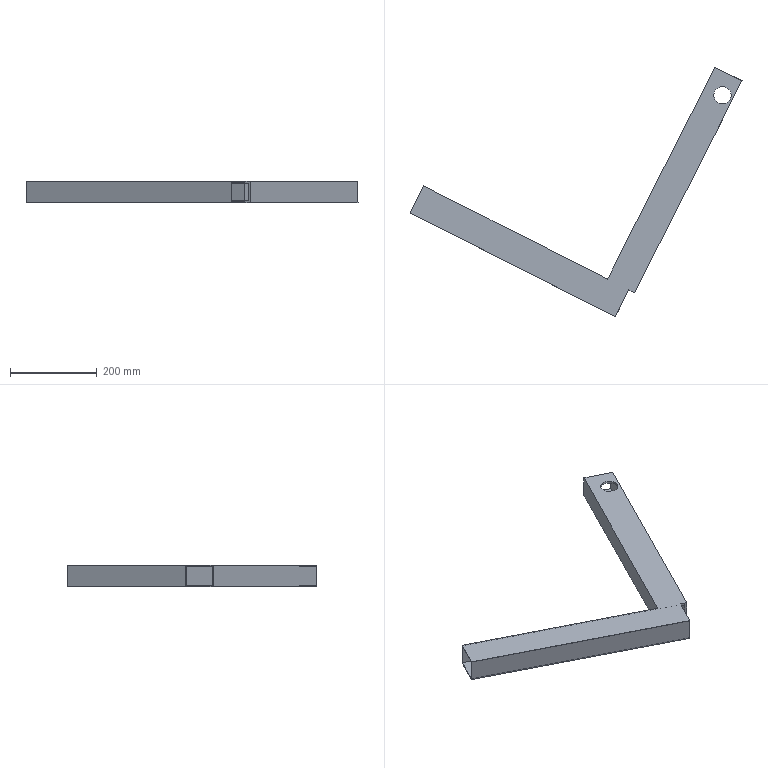Component | SolidWorks | FrameAssemblyDrawing11111-1_Part6-1 | 1 solid | 23 faces | box 765.52 x 576.1 x 50 mm | volume 836154 mm3 | plane 19 | cylinder 4 | commonest cylinder face diameters 40 x4
build123d program:
from build123d import *

# Parameters (mm, degrees)
SKETCH1_W           = 530
SKETCH1_H           = 70
BOSS_EXTRUDE1_DEPTH = 50
SHELL1_T            = -2
SKETCH2_W           = 50
SKETCH2_H           = 70
SKETCH2_W_2         = 40
SKETCH2_H_2         = 60
BOSS_EXTRUDE2_DEPTH = 548
SKETCH3_R           = 20
CUT_EXTRUDE1_DEPTH  = 779.905


with BuildPart() as part:
    # Sketch1 → Boss-Extrude1 (new body)
    with BuildSketch(Plane(origin=(0, 0, 0), x_dir=(0, 0, -1), z_dir=(1, 0, 0))):
        with Locations((198.067, 29.899)):
            Rectangle(SKETCH1_W, SKETCH1_H)
    extrude(amount=BOSS_EXTRUDE1_DEPTH)

    # Shell1
    shell1_openings = [part.faces().sort_by_distance(p)[0] for p in [
        (25, 29.899, -463.067),
        (25, 29.899, 66.933),
    ]]
    offset(amount=SHELL1_T, openings=shell1_openings, kind=Kind.INTERSECTION)

    # Sketch2 → Boss-Extrude2 (add)
    with BuildSketch(Plane(origin=(0, 64.899, 0), x_dir=(1, 0, 0), z_dir=(0, 1, 0))):
        with Locations((25, 443.067)):
            Rectangle(SKETCH2_W, SKETCH2_H)
        with Locations((25, 443.067)):
            Rectangle(SKETCH2_W_2, SKETCH2_H_2, mode=Mode.SUBTRACT)
    extrude(amount=BOSS_EXTRUDE2_DEPTH)

    # Sketch3 → Cut-Extrude1 (cut, through all)
    with BuildSketch(Plane(origin=(50, 0, 0), x_dir=(0, 0, -1), z_dir=(1, 0, 0))):
        with Locations((453.067, 562.899)):
            Circle(SKETCH3_R)
    extrude(amount=-CUT_EXTRUDE1_DEPTH, mode=Mode.SUBTRACT)


solid = part.part

# Placed as in the assembly
solid = solid.moved(Location((-784.566, -450.583, 1035.971), (-90, -63.121, -90)))
STEP:
#1=COLOUR_RGB('',0.7922,0.8196,0.9333);
#2=FILL_AREA_STYLE_COLOUR('',#1);
#3=FILL_AREA_STYLE('',(#2));
#4=SURFACE_STYLE_FILL_AREA(#3);
#5=SURFACE_SIDE_STYLE('',(#4));
#6=SURFACE_STYLE_USAGE(.BOTH.,#5);
#7=PRESENTATION_STYLE_ASSIGNMENT((#6));
#8=CARTESIAN_POINT('',(-5.661,-5.681,40.786));
#9=VERTEX_POINT('',#8);
#10=CARTESIAN_POINT('',(-4.257,-6.392,40.786));
#11=VERTEX_POINT('',#10);
#12=CARTESIAN_POINT('',(-4.959,-6.036,40.786));
#13=DIRECTION('',(-0.,-0.,1.));
#14=DIRECTION('',(0.892,-0.4521,-0.));
#15=AXIS2_PLACEMENT_3D('',#12,#13,#14);
#16=CIRCLE('',#15,0.7874);
#17=EDGE_CURVE('',#9,#11,#16,.T.);
#18=ORIENTED_EDGE('',*,*,#17,.F.);
#19=CARTESIAN_POINT('',(-5.661,-5.681,40.983));
#20=VERTEX_POINT('',#19);
#21=CARTESIAN_POINT('',(-5.661,-5.681,40.786));
#22=DIRECTION('',(-0.,-0.,1.));
#23=VECTOR('',#22,39.37);
#24=LINE('',#21,#23);
#25=EDGE_CURVE('',#9,#20,#24,.T.);
#26=ORIENTED_EDGE('',*,*,#25,.T.);
#27=CARTESIAN_POINT('',(-4.257,-6.392,40.983));
#28=VERTEX_POINT('',#27);
#29=CARTESIAN_POINT('',(-4.959,-6.036,40.983));
#30=DIRECTION('',(-0.,-0.,1.));
#31=DIRECTION('',(0.892,-0.4521,-0.));
#32=AXIS2_PLACEMENT_3D('',#29,#30,#31);
#33=CIRCLE('',#32,0.7874);
#34=EDGE_CURVE('',#20,#28,#33,.T.);
#35=ORIENTED_EDGE('',*,*,#34,.T.);
#36=CARTESIAN_POINT('',(-4.257,-6.392,40.786));
#37=DIRECTION('',(-0.,-0.,1.));
#38=VECTOR('',#37,39.37);
#39=LINE('',#36,#38);
#40=EDGE_CURVE('',#11,#28,#39,.T.);
#41=ORIENTED_EDGE('',*,*,#40,.F.);
#42=EDGE_LOOP('',(#18,#26,#35,#41));
#43=FACE_OUTER_BOUND('',#42,.T.);
#44=CARTESIAN_POINT('',(-4.959,-6.036,40.786));
#45=DIRECTION('',(-0.,-0.,1.));
#46=DIRECTION('',(0.892,-0.4521,-0.));
#47=AXIS2_PLACEMENT_3D('',#44,#45,#46);
#48=CYLINDRICAL_SURFACE('',#47,0.7874);
#49=ADVANCED_FACE('',(#43),#48,.F.);
#50=CARTESIAN_POINT('',(-4.257,-6.392,42.558));
#51=VERTEX_POINT('',#50);
#52=CARTESIAN_POINT('',(-5.661,-5.681,42.558));
#53=VERTEX_POINT('',#52);
#54=CARTESIAN_POINT('',(-4.959,-6.036,42.558));
#55=DIRECTION('',(0.,0.,-1.));
#56=DIRECTION('',(-0.892,0.4521,0.));
#57=AXIS2_PLACEMENT_3D('',#54,#55,#56);
#58=CIRCLE('',#57,0.7874);
#59=EDGE_CURVE('',#51,#53,#58,.T.);
#60=ORIENTED_EDGE('',*,*,#59,.T.);
#61=CARTESIAN_POINT('',(-5.661,-5.681,42.755));
#62=VERTEX_POINT('',#61);
#63=CARTESIAN_POINT('',(-5.661,-5.681,40.786));
#64=DIRECTION('',(-0.,-0.,1.));
#65=VECTOR('',#64,39.37);
#66=LINE('',#63,#65);
#67=EDGE_CURVE('',#53,#62,#66,.T.);
#68=ORIENTED_EDGE('',*,*,#67,.T.);
#69=CARTESIAN_POINT('',(-4.257,-6.392,42.755));
#70=VERTEX_POINT('',#69);
#71=CARTESIAN_POINT('',(-4.959,-6.036,42.755));
#72=DIRECTION('',(-0.,-0.,1.));
#73=DIRECTION('',(0.892,-0.4521,-0.));
#74=AXIS2_PLACEMENT_3D('',#71,#72,#73);
#75=CIRCLE('',#74,0.7874);
#76=EDGE_CURVE('',#62,#70,#75,.T.);
#77=ORIENTED_EDGE('',*,*,#76,.T.);
#78=CARTESIAN_POINT('',(-4.257,-6.392,40.786));
#79=DIRECTION('',(-0.,-0.,1.));
#80=VECTOR('',#79,39.37);
#81=LINE('',#78,#80);
#82=EDGE_CURVE('',#51,#70,#81,.T.);
#83=ORIENTED_EDGE('',*,*,#82,.F.);
#84=EDGE_LOOP('',(#60,#68,#77,#83));
#85=FACE_OUTER_BOUND('',#84,.T.);
#86=CARTESIAN_POINT('',(-4.959,-6.036,40.786));
#87=DIRECTION('',(-0.,-0.,1.));
#88=DIRECTION('',(0.892,-0.4521,-0.));
#89=AXIS2_PLACEMENT_3D('',#86,#87,#88);
#90=CYLINDRICAL_SURFACE('',#89,0.7874);
#91=ADVANCED_FACE('',(#85),#90,.F.);
#92=CARTESIAN_POINT('',(-15.403,-22.724,40.786));
#93=VERTEX_POINT('',#92);
#94=CARTESIAN_POINT('',(-15.403,-22.724,42.755));
#95=VERTEX_POINT('',#94);
#96=CARTESIAN_POINT('',(-15.403,-22.724,40.786));
#97=DIRECTION('',(-0.,-0.,1.));
#98=VECTOR('',#97,39.37);
#99=LINE('',#96,#98);
#100=EDGE_CURVE('',#93,#95,#99,.T.);
#101=ORIENTED_EDGE('',*,*,#100,.F.);
#102=CARTESIAN_POINT('',(-32.084,-14.269,40.786));
#103=VERTEX_POINT('',#102);
#104=CARTESIAN_POINT('',(-32.084,-14.269,40.786));
#105=DIRECTION('',(-0.892,0.4521,0.));
#106=VECTOR('',#105,39.37);
#107=LINE('',#104,#106);
#108=EDGE_CURVE('',#93,#103,#107,.T.);
#109=ORIENTED_EDGE('',*,*,#108,.T.);
#110=CARTESIAN_POINT('',(-32.084,-14.269,42.755));
#111=VERTEX_POINT('',#110);
#112=CARTESIAN_POINT('',(-32.084,-14.269,42.755));
#113=DIRECTION('',(0.,0.,-1.));
#114=VECTOR('',#113,39.37);
#115=LINE('',#112,#114);
#116=EDGE_CURVE('',#111,#103,#115,.T.);
#117=ORIENTED_EDGE('',*,*,#116,.F.);
#118=CARTESIAN_POINT('',(-32.084,-14.269,42.755));
#119=DIRECTION('',(-0.892,0.4521,0.));
#120=VECTOR('',#119,39.37);
#121=LINE('',#118,#120);
#122=EDGE_CURVE('',#95,#111,#121,.T.);
#123=ORIENTED_EDGE('',*,*,#122,.F.);
#124=EDGE_LOOP('',(#101,#109,#117,#123));
#125=FACE_OUTER_BOUND('',#124,.T.);
#126=CARTESIAN_POINT('',(-32.084,-14.269,42.755));
#127=DIRECTION('',(-0.4521,-0.892,-0.));
#128=DIRECTION('',(0.892,-0.4521,-0.));
#129=AXIS2_PLACEMENT_3D('',#126,#127,#128);
#130=PLANE('',#129);
#131=ADVANCED_FACE('',(#125),#130,.F.);
#132=CARTESIAN_POINT('',(-33.33,-16.727,40.786));
#133=VERTEX_POINT('',#132);
#134=CARTESIAN_POINT('',(-32.084,-14.269,40.786));
#135=DIRECTION('',(-0.4521,-0.892,-0.));
#136=VECTOR('',#135,39.37);
#137=LINE('',#134,#136);
#138=EDGE_CURVE('',#103,#133,#137,.T.);
#139=ORIENTED_EDGE('',*,*,#138,.T.);
#140=CARTESIAN_POINT('',(-33.33,-16.727,42.755));
#141=VERTEX_POINT('',#140);
#142=CARTESIAN_POINT('',(-33.33,-16.727,42.755));
#143=DIRECTION('',(0.,0.,-1.));
#144=VECTOR('',#143,39.37);
#145=LINE('',#142,#144);
#146=EDGE_CURVE('',#141,#133,#145,.T.);
#147=ORIENTED_EDGE('',*,*,#146,.F.);
#148=CARTESIAN_POINT('',(-32.084,-14.269,42.755));
#149=DIRECTION('',(-0.4521,-0.892,-0.));
#150=VECTOR('',#149,39.37);
#151=LINE('',#148,#150);
#152=EDGE_CURVE('',#111,#141,#151,.T.);
#153=ORIENTED_EDGE('',*,*,#152,.F.);
#154=ORIENTED_EDGE('',*,*,#116,.T.);
#155=EDGE_LOOP('',(#139,#147,#153,#154));
#156=FACE_OUTER_BOUND('',#155,.T.);
#157=CARTESIAN_POINT('',(-32.119,-14.339,40.865));
#158=VERTEX_POINT('',#157);
#159=CARTESIAN_POINT('',(-33.294,-16.657,40.865));
#160=VERTEX_POINT('',#159);
#161=CARTESIAN_POINT('',(-32.084,-14.269,40.865));
#162=DIRECTION('',(-0.4521,-0.892,-0.));
#163=VECTOR('',#162,39.37);
#164=LINE('',#161,#163);
#165=EDGE_CURVE('',#158,#160,#164,.T.);
#166=ORIENTED_EDGE('',*,*,#165,.F.);
#167=CARTESIAN_POINT('',(-32.119,-14.339,42.676));
#168=VERTEX_POINT('',#167);
#169=CARTESIAN_POINT('',(-32.119,-14.339,42.755));
#170=DIRECTION('',(0.,0.,-1.));
#171=VECTOR('',#170,39.37);
#172=LINE('',#169,#171);
#173=EDGE_CURVE('',#168,#158,#172,.T.);
#174=ORIENTED_EDGE('',*,*,#173,.F.);
#175=CARTESIAN_POINT('',(-33.294,-16.657,42.676));
#176=VERTEX_POINT('',#175);
#177=CARTESIAN_POINT('',(-32.084,-14.269,42.676));
#178=DIRECTION('',(-0.4521,-0.892,-0.));
#179=VECTOR('',#178,39.37);
#180=LINE('',#177,#179);
#181=EDGE_CURVE('',#168,#176,#180,.T.);
#182=ORIENTED_EDGE('',*,*,#181,.T.);
#183=CARTESIAN_POINT('',(-33.294,-16.657,42.755));
#184=DIRECTION('',(0.,0.,-1.));
#185=VECTOR('',#184,39.37);
#186=LINE('',#183,#185);
#187=EDGE_CURVE('',#176,#160,#186,.T.);
#188=ORIENTED_EDGE('',*,*,#187,.T.);
#189=EDGE_LOOP('',(#166,#174,#182,#188));
#190=FACE_BOUND('',#189,.T.);
#191=CARTESIAN_POINT('',(-32.084,-14.269,42.755));
#192=DIRECTION('',(0.892,-0.4521,-0.));
#193=DIRECTION('',(0.4521,0.892,0.));
#194=AXIS2_PLACEMENT_3D('',#191,#192,#193);
#195=PLANE('',#194);
#196=ADVANCED_FACE('',(#156,#190),#195,.F.);
#197=CARTESIAN_POINT('',(-14.718,-26.161,40.786));
#198=VERTEX_POINT('',#197);
#199=CARTESIAN_POINT('',(-13.472,-23.703,40.786));
#200=VERTEX_POINT('',#199);
#201=CARTESIAN_POINT('',(-13.472,-23.703,40.786));
#202=DIRECTION('',(0.4521,0.892,0.));
#203=VECTOR('',#202,39.37);
#204=LINE('',#201,#203);
#205=EDGE_CURVE('',#198,#200,#204,.T.);
#206=ORIENTED_EDGE('',*,*,#205,.T.);
#207=CARTESIAN_POINT('',(-13.472,-23.703,40.983));
#208=VERTEX_POINT('',#207);
#209=CARTESIAN_POINT('',(-13.472,-23.703,42.755));
#210=DIRECTION('',(0.,0.,-1.));
#211=VECTOR('',#210,39.37);
#212=LINE('',#209,#211);
#213=EDGE_CURVE('',#208,#200,#212,.T.);
#214=ORIENTED_EDGE('',*,*,#213,.F.);
#215=CARTESIAN_POINT('',(-13.472,-23.703,42.558));
#216=VERTEX_POINT('',#215);
#217=CARTESIAN_POINT('',(-13.472,-23.703,42.755));
#218=DIRECTION('',(0.,0.,-1.));
#219=VECTOR('',#218,39.37);
#220=LINE('',#217,#219);
#221=EDGE_CURVE('',#216,#208,#220,.T.);
#222=ORIENTED_EDGE('',*,*,#221,.F.);
#223=CARTESIAN_POINT('',(-13.472,-23.703,42.755));
#224=VERTEX_POINT('',#223);
#225=CARTESIAN_POINT('',(-13.472,-23.703,42.755));
#226=DIRECTION('',(0.,0.,-1.));
#227=VECTOR('',#226,39.37);
#228=LINE('',#225,#227);
#229=EDGE_CURVE('',#224,#216,#228,.T.);
#230=ORIENTED_EDGE('',*,*,#229,.F.);
#231=CARTESIAN_POINT('',(-14.718,-26.161,42.755));
#232=VERTEX_POINT('',#231);
#233=CARTESIAN_POINT('',(-13.472,-23.703,42.755));
#234=DIRECTION('',(0.4521,0.892,0.));
#235=VECTOR('',#234,39.37);
#236=LINE('',#233,#235);
#237=EDGE_CURVE('',#232,#224,#236,.T.);
#238=ORIENTED_EDGE('',*,*,#237,.F.);
#239=CARTESIAN_POINT('',(-14.718,-26.161,42.755));
#240=DIRECTION('',(0.,0.,-1.));
#241=VECTOR('',#240,39.37);
#242=LINE('',#239,#241);
#243=EDGE_CURVE('',#232,#198,#242,.T.);
#244=ORIENTED_EDGE('',*,*,#243,.T.);
#245=EDGE_LOOP('',(#206,#214,#222,#230,#238,#244));
#246=FACE_OUTER_BOUND('',#245,.T.);
#247=CARTESIAN_POINT('',(-14.682,-26.091,40.865));
#248=VERTEX_POINT('',#247);
#249=CARTESIAN_POINT('',(-13.507,-23.773,40.865));
#250=VERTEX_POINT('',#249);
#251=CARTESIAN_POINT('',(-13.472,-23.703,40.865));
#252=DIRECTION('',(0.4521,0.892,0.));
#253=VECTOR('',#252,39.37);
#254=LINE('',#251,#253);
#255=EDGE_CURVE('',#248,#250,#254,.T.);
#256=ORIENTED_EDGE('',*,*,#255,.F.);
#257=CARTESIAN_POINT('',(-14.682,-26.091,42.676));
#258=VERTEX_POINT('',#257);
#259=CARTESIAN_POINT('',(-14.682,-26.091,42.755));
#260=DIRECTION('',(0.,0.,-1.));
#261=VECTOR('',#260,39.37);
#262=LINE('',#259,#261);
#263=EDGE_CURVE('',#258,#248,#262,.T.);
#264=ORIENTED_EDGE('',*,*,#263,.F.);
#265=CARTESIAN_POINT('',(-13.507,-23.773,42.676));
#266=VERTEX_POINT('',#265);
#267=CARTESIAN_POINT('',(-13.472,-23.703,42.676));
#268=DIRECTION('',(0.4521,0.892,0.));
#269=VECTOR('',#268,39.37);
#270=LINE('',#267,#269);
#271=EDGE_CURVE('',#258,#266,#270,.T.);
#272=ORIENTED_EDGE('',*,*,#271,.T.);
#273=CARTESIAN_POINT('',(-13.507,-23.773,42.755));
#274=DIRECTION('',(0.,0.,-1.));
#275=VECTOR('',#274,39.37);
#276=LINE('',#273,#275);
#277=EDGE_CURVE('',#266,#250,#276,.T.);
#278=ORIENTED_EDGE('',*,*,#277,.T.);
#279=EDGE_LOOP('',(#256,#264,#272,#278));
#280=FACE_BOUND('',#279,.T.);
#281=CARTESIAN_POINT('',(-13.472,-23.703,42.755));
#282=DIRECTION('',(-0.892,0.4521,0.));
#283=DIRECTION('',(-0.,-0.,1.));
#284=AXIS2_PLACEMENT_3D('',#281,#282,#283);
#285=PLANE('',#284);
#286=ADVANCED_FACE('',(#246,#280),#285,.F.);
#287=CARTESIAN_POINT('',(-33.33,-16.727,40.786));
#288=DIRECTION('',(0.892,-0.4521,-0.));
#289=VECTOR('',#288,39.37);
#290=LINE('',#287,#289);
#291=EDGE_CURVE('',#133,#198,#290,.T.);
#292=ORIENTED_EDGE('',*,*,#291,.T.);
#293=ORIENTED_EDGE('',*,*,#243,.F.);
#294=CARTESIAN_POINT('',(-33.33,-16.727,42.755));
#295=DIRECTION('',(0.892,-0.4521,-0.));
#296=VECTOR('',#295,39.37);
#297=LINE('',#294,#296);
#298=EDGE_CURVE('',#141,#232,#297,.T.);
#299=ORIENTED_EDGE('',*,*,#298,.F.);
#300=ORIENTED_EDGE('',*,*,#146,.T.);
#301=EDGE_LOOP('',(#292,#293,#299,#300));
#302=FACE_OUTER_BOUND('',#301,.T.);
#303=CARTESIAN_POINT('',(-33.33,-16.727,42.755));
#304=DIRECTION('',(0.4521,0.892,0.));
#305=DIRECTION('',(-0.892,0.4521,0.));
#306=AXIS2_PLACEMENT_3D('',#303,#304,#305);
#307=PLANE('',#306);
#308=ADVANCED_FACE('',(#302),#307,.F.);
#309=ORIENTED_EDGE('',*,*,#221,.T.);
#310=CARTESIAN_POINT('',(-15.228,-22.813,40.983));
#311=VERTEX_POINT('',#310);
#312=CARTESIAN_POINT('',(-13.121,-23.881,40.983));
#313=DIRECTION('',(-0.892,0.4521,0.));
#314=VECTOR('',#313,39.37);
#315=LINE('',#312,#314);
#316=EDGE_CURVE('',#208,#311,#315,.T.);
#317=ORIENTED_EDGE('',*,*,#316,.T.);
#318=CARTESIAN_POINT('',(-15.228,-22.813,42.558));
#319=VERTEX_POINT('',#318);
#320=CARTESIAN_POINT('',(-15.228,-22.813,40.983));
#321=DIRECTION('',(-0.,-0.,1.));
#322=VECTOR('',#321,39.37);
#323=LINE('',#320,#322);
#324=EDGE_CURVE('',#311,#319,#323,.T.);
#325=ORIENTED_EDGE('',*,*,#324,.T.);
#326=CARTESIAN_POINT('',(-13.121,-23.881,42.558));
#327=DIRECTION('',(0.892,-0.4521,-0.));
#328=VECTOR('',#327,39.37);
#329=LINE('',#326,#328);
#330=EDGE_CURVE('',#319,#216,#329,.T.);
#331=ORIENTED_EDGE('',*,*,#330,.T.);
#332=EDGE_LOOP('',(#309,#317,#325,#331));
#333=FACE_OUTER_BOUND('',#332,.T.);
#334=CARTESIAN_POINT('',(-32.084,-14.269,42.755));
#335=DIRECTION('',(-0.4521,-0.892,-0.));
#336=DIRECTION('',(0.892,-0.4521,-0.));
#337=AXIS2_PLACEMENT_3D('',#334,#335,#336);
#338=PLANE('',#337);
#339=ADVANCED_FACE('',(#333),#338,.F.);
#340=CARTESIAN_POINT('',(-4.959,-6.036,42.755));
#341=DIRECTION('',(-0.,-0.,1.));
#342=DIRECTION('',(0.892,-0.4521,-0.));
#343=AXIS2_PLACEMENT_3D('',#340,#341,#342);
#344=CIRCLE('',#343,0.7874);
#345=EDGE_CURVE('',#70,#62,#344,.T.);
#346=ORIENTED_EDGE('',*,*,#345,.F.);
#347=ORIENTED_EDGE('',*,*,#76,.F.);
#348=EDGE_LOOP('',(#346,#347));
#349=FACE_BOUND('',#348,.T.);
#350=ORIENTED_EDGE('',*,*,#152,.T.);
#351=ORIENTED_EDGE('',*,*,#298,.T.);
#352=ORIENTED_EDGE('',*,*,#237,.T.);
#353=CARTESIAN_POINT('',(-12.945,-23.97,42.755));
#354=VERTEX_POINT('',#353);
#355=CARTESIAN_POINT('',(-12.945,-23.97,42.755));
#356=DIRECTION('',(0.892,-0.4521,-0.));
#357=VECTOR('',#356,39.37);
#358=LINE('',#355,#357);
#359=EDGE_CURVE('',#224,#354,#358,.T.);
#360=ORIENTED_EDGE('',*,*,#359,.T.);
#361=CARTESIAN_POINT('',(-3.191,-4.726,42.755));
#362=VERTEX_POINT('',#361);
#363=CARTESIAN_POINT('',(-3.191,-4.726,42.755));
#364=DIRECTION('',(-0.4521,-0.892,-0.));
#365=VECTOR('',#364,39.37);
#366=LINE('',#363,#365);
#367=EDGE_CURVE('',#362,#354,#366,.T.);
#368=ORIENTED_EDGE('',*,*,#367,.F.);
#369=CARTESIAN_POINT('',(-5.649,-3.48,42.755));
#370=VERTEX_POINT('',#369);
#371=CARTESIAN_POINT('',(-3.191,-4.726,42.755));
#372=DIRECTION('',(0.892,-0.4521,-0.));
#373=VECTOR('',#372,39.37);
#374=LINE('',#371,#373);
#375=EDGE_CURVE('',#370,#362,#374,.T.);
#376=ORIENTED_EDGE('',*,*,#375,.F.);
#377=CARTESIAN_POINT('',(-5.649,-3.48,42.755));
#378=DIRECTION('',(-0.4521,-0.892,-0.));
#379=VECTOR('',#378,39.37);
#380=LINE('',#377,#379);
#381=EDGE_CURVE('',#370,#95,#380,.T.);
#382=ORIENTED_EDGE('',*,*,#381,.T.);
#383=ORIENTED_EDGE('',*,*,#122,.T.);
#384=EDGE_LOOP('',(#350,#351,#352,#360,#368,#376,#382,#383));
#385=FACE_OUTER_BOUND('',#384,.T.);
#386=CARTESIAN_POINT('',(-30.888,-17.739,42.755));
#387=DIRECTION('',(-0.,-0.,1.));
#388=DIRECTION('',(0.892,-0.4521,-0.));
#389=AXIS2_PLACEMENT_3D('',#386,#387,#388);
#390=PLANE('',#389);
#391=ADVANCED_FACE('',(#349,#385),#390,.T.);
#392=CARTESIAN_POINT('',(-4.959,-6.036,40.786));
#393=DIRECTION('',(-0.,-0.,1.));
#394=DIRECTION('',(0.892,-0.4521,-0.));
#395=AXIS2_PLACEMENT_3D('',#392,#393,#394);
#396=CIRCLE('',#395,0.7874);
#397=EDGE_CURVE('',#11,#9,#396,.T.);
#398=ORIENTED_EDGE('',*,*,#397,.T.);
#399=ORIENTED_EDGE('',*,*,#17,.T.);
#400=EDGE_LOOP('',(#398,#399));
#401=FACE_BOUND('',#400,.T.);
#402=ORIENTED_EDGE('',*,*,#138,.F.);
#403=ORIENTED_EDGE('',*,*,#108,.F.);
#404=CARTESIAN_POINT('',(-5.649,-3.48,40.786));
#405=VERTEX_POINT('',#404);
#406=CARTESIAN_POINT('',(-5.649,-3.48,40.786));
#407=DIRECTION('',(-0.4521,-0.892,-0.));
#408=VECTOR('',#407,39.37);
#409=LINE('',#406,#408);
#410=EDGE_CURVE('',#405,#93,#409,.T.);
#411=ORIENTED_EDGE('',*,*,#410,.F.);
#412=CARTESIAN_POINT('',(-3.191,-4.726,40.786));
#413=VERTEX_POINT('',#412);
#414=CARTESIAN_POINT('',(-3.191,-4.726,40.786));
#415=DIRECTION('',(-0.892,0.4521,0.));
#416=VECTOR('',#415,39.37);
#417=LINE('',#414,#416);
#418=EDGE_CURVE('',#413,#405,#417,.T.);
#419=ORIENTED_EDGE('',*,*,#418,.F.);
#420=CARTESIAN_POINT('',(-12.945,-23.97,40.786));
#421=VERTEX_POINT('',#420);
#422=CARTESIAN_POINT('',(-3.191,-4.726,40.786));
#423=DIRECTION('',(-0.4521,-0.892,-0.));
#424=VECTOR('',#423,39.37);
#425=LINE('',#422,#424);
#426=EDGE_CURVE('',#413,#421,#425,.T.);
#427=ORIENTED_EDGE('',*,*,#426,.T.);
#428=CARTESIAN_POINT('',(-12.945,-23.97,40.786));
#429=DIRECTION('',(-0.892,0.4521,0.));
#430=VECTOR('',#429,39.37);
#431=LINE('',#428,#430);
#432=EDGE_CURVE('',#421,#200,#431,.T.);
#433=ORIENTED_EDGE('',*,*,#432,.T.);
#434=ORIENTED_EDGE('',*,*,#205,.F.);
#435=ORIENTED_EDGE('',*,*,#291,.F.);
#436=EDGE_LOOP('',(#402,#403,#411,#419,#427,#433,#434,#435));
#437=FACE_OUTER_BOUND('',#436,.T.);
#438=CARTESIAN_POINT('',(-30.888,-17.739,40.786));
#439=DIRECTION('',(-0.,-0.,1.));
#440=DIRECTION('',(0.892,-0.4521,-0.));
#441=AXIS2_PLACEMENT_3D('',#438,#439,#440);
#442=PLANE('',#441);
#443=ADVANCED_FACE('',(#401,#437),#442,.F.);
#444=CARTESIAN_POINT('',(-33.294,-16.657,40.865));
#445=DIRECTION('',(0.892,-0.4521,-0.));
#446=VECTOR('',#445,39.37);
#447=LINE('',#444,#446);
#448=EDGE_CURVE('',#160,#248,#447,.T.);
#449=ORIENTED_EDGE('',*,*,#448,.F.);
#450=ORIENTED_EDGE('',*,*,#187,.F.);
#451=CARTESIAN_POINT('',(-33.294,-16.657,42.676));
#452=DIRECTION('',(0.892,-0.4521,-0.));
#453=VECTOR('',#452,39.37);
#454=LINE('',#451,#453);
#455=EDGE_CURVE('',#176,#258,#454,.T.);
#456=ORIENTED_EDGE('',*,*,#455,.T.);
#457=ORIENTED_EDGE('',*,*,#263,.T.);
#458=EDGE_LOOP('',(#449,#450,#456,#457));
#459=FACE_OUTER_BOUND('',#458,.T.);
#460=CARTESIAN_POINT('',(-33.294,-16.657,42.755));
#461=DIRECTION('',(0.4521,0.892,0.));
#462=DIRECTION('',(-0.892,0.4521,0.));
#463=AXIS2_PLACEMENT_3D('',#460,#461,#462);
#464=PLANE('',#463);
#465=ADVANCED_FACE('',(#459),#464,.T.);
#466=CARTESIAN_POINT('',(-32.119,-14.339,40.865));
#467=DIRECTION('',(-0.892,0.4521,0.));
#468=VECTOR('',#467,39.37);
#469=LINE('',#466,#468);
#470=EDGE_CURVE('',#250,#158,#469,.T.);
#471=ORIENTED_EDGE('',*,*,#470,.F.);
#472=ORIENTED_EDGE('',*,*,#277,.F.);
#473=CARTESIAN_POINT('',(-32.119,-14.339,42.676));
#474=DIRECTION('',(-0.892,0.4521,0.));
#475=VECTOR('',#474,39.37);
#476=LINE('',#473,#475);
#477=EDGE_CURVE('',#266,#168,#476,.T.);
#478=ORIENTED_EDGE('',*,*,#477,.T.);
#479=ORIENTED_EDGE('',*,*,#173,.T.);
#480=EDGE_LOOP('',(#471,#472,#478,#479));
#481=FACE_OUTER_BOUND('',#480,.T.);
#482=CARTESIAN_POINT('',(-32.119,-14.339,42.755));
#483=DIRECTION('',(-0.4521,-0.892,-0.));
#484=DIRECTION('',(0.892,-0.4521,-0.));
#485=AXIS2_PLACEMENT_3D('',#482,#483,#484);
#486=PLANE('',#485);
#487=ADVANCED_FACE('',(#481),#486,.T.);
#488=ORIENTED_EDGE('',*,*,#181,.F.);
#489=ORIENTED_EDGE('',*,*,#477,.F.);
#490=ORIENTED_EDGE('',*,*,#271,.F.);
#491=ORIENTED_EDGE('',*,*,#455,.F.);
#492=EDGE_LOOP('',(#488,#489,#490,#491));
#493=FACE_OUTER_BOUND('',#492,.T.);
#494=CARTESIAN_POINT('',(-30.888,-17.739,42.676));
#495=DIRECTION('',(-0.,-0.,1.));
#496=DIRECTION('',(0.892,-0.4521,-0.));
#497=AXIS2_PLACEMENT_3D('',#494,#495,#496);
#498=PLANE('',#497);
#499=ADVANCED_FACE('',(#493),#498,.F.);
#500=ORIENTED_EDGE('',*,*,#165,.T.);
#501=ORIENTED_EDGE('',*,*,#448,.T.);
#502=ORIENTED_EDGE('',*,*,#255,.T.);
#503=ORIENTED_EDGE('',*,*,#470,.T.);
#504=EDGE_LOOP('',(#500,#501,#502,#503));
#505=FACE_OUTER_BOUND('',#504,.T.);
#506=CARTESIAN_POINT('',(-30.888,-17.739,40.865));
#507=DIRECTION('',(-0.,-0.,1.));
#508=DIRECTION('',(0.892,-0.4521,-0.));
#509=AXIS2_PLACEMENT_3D('',#506,#507,#508);
#510=PLANE('',#509);
#511=ADVANCED_FACE('',(#505),#510,.T.);
#512=ORIENTED_EDGE('',*,*,#359,.F.);
#513=ORIENTED_EDGE('',*,*,#229,.T.);
#514=CARTESIAN_POINT('',(-13.121,-23.881,42.558));
#515=VERTEX_POINT('',#514);
#516=CARTESIAN_POINT('',(-13.121,-23.881,42.558));
#517=DIRECTION('',(0.892,-0.4521,-0.));
#518=VECTOR('',#517,39.37);
#519=LINE('',#516,#518);
#520=EDGE_CURVE('',#216,#515,#519,.T.);
#521=ORIENTED_EDGE('',*,*,#520,.T.);
#522=CARTESIAN_POINT('',(-13.121,-23.881,40.983));
#523=VERTEX_POINT('',#522);
#524=CARTESIAN_POINT('',(-13.121,-23.881,40.983));
#525=DIRECTION('',(0.,0.,-1.));
#526=VECTOR('',#525,39.37);
#527=LINE('',#524,#526);
#528=EDGE_CURVE('',#515,#523,#527,.T.);
#529=ORIENTED_EDGE('',*,*,#528,.T.);
#530=CARTESIAN_POINT('',(-13.121,-23.881,40.983));
#531=DIRECTION('',(-0.892,0.4521,0.));
#532=VECTOR('',#531,39.37);
#533=LINE('',#530,#532);
#534=EDGE_CURVE('',#523,#208,#533,.T.);
#535=ORIENTED_EDGE('',*,*,#534,.T.);
#536=ORIENTED_EDGE('',*,*,#213,.T.);
#537=ORIENTED_EDGE('',*,*,#432,.F.);
#538=CARTESIAN_POINT('',(-12.945,-23.97,40.786));
#539=DIRECTION('',(0.,0.,-1.));
#540=VECTOR('',#539,39.37);
#541=LINE('',#538,#540);
#542=EDGE_CURVE('',#354,#421,#541,.T.);
#543=ORIENTED_EDGE('',*,*,#542,.F.);
#544=EDGE_LOOP('',(#512,#513,#521,#529,#535,#536,#537,#543));
#545=FACE_OUTER_BOUND('',#544,.T.);
#546=CARTESIAN_POINT('',(-29.733,-15.46,40.786));
#547=DIRECTION('',(0.4521,0.892,0.));
#548=DIRECTION('',(-0.892,0.4521,0.));
#549=AXIS2_PLACEMENT_3D('',#546,#547,#548);
#550=PLANE('',#549);
#551=ADVANCED_FACE('',(#545),#550,.F.);
#552=ORIENTED_EDGE('',*,*,#418,.T.);
#553=CARTESIAN_POINT('',(-5.649,-3.48,40.786));
#554=DIRECTION('',(-0.,-0.,1.));
#555=VECTOR('',#554,39.37);
#556=LINE('',#553,#555);
#557=EDGE_CURVE('',#405,#370,#556,.T.);
#558=ORIENTED_EDGE('',*,*,#557,.T.);
#559=ORIENTED_EDGE('',*,*,#375,.T.);
#560=CARTESIAN_POINT('',(-3.191,-4.726,40.786));
#561=DIRECTION('',(0.,0.,-1.));
#562=VECTOR('',#561,39.37);
#563=LINE('',#560,#562);
#564=EDGE_CURVE('',#362,#413,#563,.T.);
#565=ORIENTED_EDGE('',*,*,#564,.T.);
#566=EDGE_LOOP('',(#552,#558,#559,#565));
#567=FACE_OUTER_BOUND('',#566,.T.);
#568=CARTESIAN_POINT('',(-5.474,-3.569,40.983));
#569=VERTEX_POINT('',#568);
#570=CARTESIAN_POINT('',(-5.474,-3.569,42.558));
#571=VERTEX_POINT('',#570);
#572=CARTESIAN_POINT('',(-5.474,-3.569,40.983));
#573=DIRECTION('',(-0.,-0.,1.));
#574=VECTOR('',#573,39.37);
#575=LINE('',#572,#574);
#576=EDGE_CURVE('',#569,#571,#575,.T.);
#577=ORIENTED_EDGE('',*,*,#576,.F.);
#578=CARTESIAN_POINT('',(-3.367,-4.637,40.983));
#579=VERTEX_POINT('',#578);
#580=CARTESIAN_POINT('',(-3.367,-4.637,40.983));
#581=DIRECTION('',(-0.892,0.4521,0.));
#582=VECTOR('',#581,39.37);
#583=LINE('',#580,#582);
#584=EDGE_CURVE('',#579,#569,#583,.T.);
#585=ORIENTED_EDGE('',*,*,#584,.F.);
#586=CARTESIAN_POINT('',(-3.367,-4.637,42.558));
#587=VERTEX_POINT('',#586);
#588=CARTESIAN_POINT('',(-3.367,-4.637,40.983));
#589=DIRECTION('',(0.,0.,-1.));
#590=VECTOR('',#589,39.37);
#591=LINE('',#588,#590);
#592=EDGE_CURVE('',#587,#579,#591,.T.);
#593=ORIENTED_EDGE('',*,*,#592,.F.);
#594=CARTESIAN_POINT('',(-3.367,-4.637,42.558));
#595=DIRECTION('',(0.892,-0.4521,-0.));
#596=VECTOR('',#595,39.37);
#597=LINE('',#594,#596);
#598=EDGE_CURVE('',#571,#587,#597,.T.);
#599=ORIENTED_EDGE('',*,*,#598,.F.);
#600=EDGE_LOOP('',(#577,#585,#593,#599));
#601=FACE_BOUND('',#600,.T.);
#602=CARTESIAN_POINT('',(-19.979,3.784,40.786));
#603=DIRECTION('',(0.4521,0.892,0.));
#604=DIRECTION('',(-0.892,0.4521,0.));
#605=AXIS2_PLACEMENT_3D('',#602,#603,#604);
#606=PLANE('',#605);
#607=ADVANCED_FACE('',(#567,#601),#606,.T.);
#608=ORIENTED_EDGE('',*,*,#100,.T.);
#609=ORIENTED_EDGE('',*,*,#381,.F.);
#610=ORIENTED_EDGE('',*,*,#557,.F.);
#611=ORIENTED_EDGE('',*,*,#410,.T.);
#612=EDGE_LOOP('',(#608,#609,#610,#611));
#613=FACE_OUTER_BOUND('',#612,.T.);
#614=CARTESIAN_POINT('',(-5.649,-3.48,40.786));
#615=DIRECTION('',(0.892,-0.4521,-0.));
#616=DIRECTION('',(0.,0.,-1.));
#617=AXIS2_PLACEMENT_3D('',#614,#615,#616);
#618=PLANE('',#617);
#619=ADVANCED_FACE('',(#613),#618,.F.);
#620=ORIENTED_EDGE('',*,*,#542,.T.);
#621=ORIENTED_EDGE('',*,*,#426,.F.);
#622=ORIENTED_EDGE('',*,*,#564,.F.);
#623=ORIENTED_EDGE('',*,*,#367,.T.);
#624=EDGE_LOOP('',(#620,#621,#622,#623));
#625=FACE_OUTER_BOUND('',#624,.T.);
#626=CARTESIAN_POINT('',(-3.191,-4.726,40.786));
#627=DIRECTION('',(-0.892,0.4521,0.));
#628=DIRECTION('',(-0.,-0.,1.));
#629=AXIS2_PLACEMENT_3D('',#626,#627,#628);
#630=PLANE('',#629);
#631=ADVANCED_FACE('',(#625),#630,.F.);
#632=CARTESIAN_POINT('',(-3.367,-4.637,40.983));
#633=DIRECTION('',(-0.4521,-0.892,-0.));
#634=VECTOR('',#633,39.37);
#635=LINE('',#632,#634);
#636=EDGE_CURVE('',#28,#523,#635,.T.);
#637=ORIENTED_EDGE('',*,*,#636,.F.);
#638=ORIENTED_EDGE('',*,*,#34,.F.);
#639=CARTESIAN_POINT('',(-4.959,-6.036,40.983));
#640=DIRECTION('',(-0.,-0.,1.));
#641=DIRECTION('',(0.892,-0.4521,-0.));
#642=AXIS2_PLACEMENT_3D('',#639,#640,#641);
#643=CIRCLE('',#642,0.7874);
#644=EDGE_CURVE('',#28,#20,#643,.T.);
#645=ORIENTED_EDGE('',*,*,#644,.F.);
#646=CARTESIAN_POINT('',(-3.367,-4.637,40.983));
#647=DIRECTION('',(-0.4521,-0.892,-0.));
#648=VECTOR('',#647,39.37);
#649=LINE('',#646,#648);
#650=EDGE_CURVE('',#579,#28,#649,.T.);
#651=ORIENTED_EDGE('',*,*,#650,.F.);
#652=ORIENTED_EDGE('',*,*,#584,.T.);
#653=CARTESIAN_POINT('',(-5.474,-3.569,40.983));
#654=DIRECTION('',(-0.4521,-0.892,-0.));
#655=VECTOR('',#654,39.37);
#656=LINE('',#653,#655);
#657=EDGE_CURVE('',#569,#311,#656,.T.);
#658=ORIENTED_EDGE('',*,*,#657,.T.);
#659=ORIENTED_EDGE('',*,*,#316,.F.);
#660=ORIENTED_EDGE('',*,*,#534,.F.);
#661=EDGE_LOOP('',(#637,#638,#645,#651,#652,#658,#659,#660));
#662=FACE_OUTER_BOUND('',#661,.T.);
#663=CARTESIAN_POINT('',(-3.367,-4.637,40.983));
#664=DIRECTION('',(-0.,-0.,1.));
#665=DIRECTION('',(0.892,-0.4521,-0.));
#666=AXIS2_PLACEMENT_3D('',#663,#664,#665);
#667=PLANE('',#666);
#668=ADVANCED_FACE('',(#662),#667,.T.);
#669=ORIENTED_EDGE('',*,*,#324,.F.);
#670=ORIENTED_EDGE('',*,*,#657,.F.);
#671=ORIENTED_EDGE('',*,*,#576,.T.);
#672=CARTESIAN_POINT('',(-5.474,-3.569,42.558));
#673=DIRECTION('',(-0.4521,-0.892,-0.));
#674=VECTOR('',#673,39.37);
#675=LINE('',#672,#674);
#676=EDGE_CURVE('',#571,#319,#675,.T.);
#677=ORIENTED_EDGE('',*,*,#676,.T.);
#678=EDGE_LOOP('',(#669,#670,#671,#677));
#679=FACE_OUTER_BOUND('',#678,.T.);
#680=CARTESIAN_POINT('',(-5.474,-3.569,40.983));
#681=DIRECTION('',(0.892,-0.4521,-0.));
#682=DIRECTION('',(0.,0.,-1.));
#683=AXIS2_PLACEMENT_3D('',#680,#681,#682);
#684=PLANE('',#683);
#685=ADVANCED_FACE('',(#679),#684,.T.);
#686=CARTESIAN_POINT('',(-3.367,-4.637,42.558));
#687=DIRECTION('',(-0.4521,-0.892,-0.));
#688=VECTOR('',#687,39.37);
#689=LINE('',#686,#688);
#690=EDGE_CURVE('',#587,#51,#689,.T.);
#691=ORIENTED_EDGE('',*,*,#690,.T.);
#692=CARTESIAN_POINT('',(-4.959,-6.036,42.558));
#693=DIRECTION('',(0.,0.,-1.));
#694=DIRECTION('',(-0.892,0.4521,0.));
#695=AXIS2_PLACEMENT_3D('',#692,#693,#694);
#696=CIRCLE('',#695,0.7874);
#697=EDGE_CURVE('',#53,#51,#696,.T.);
#698=ORIENTED_EDGE('',*,*,#697,.F.);
#699=ORIENTED_EDGE('',*,*,#59,.F.);
#700=CARTESIAN_POINT('',(-3.367,-4.637,42.558));
#701=DIRECTION('',(-0.4521,-0.892,-0.));
#702=VECTOR('',#701,39.37);
#703=LINE('',#700,#702);
#704=EDGE_CURVE('',#51,#515,#703,.T.);
#705=ORIENTED_EDGE('',*,*,#704,.T.);
#706=ORIENTED_EDGE('',*,*,#520,.F.);
#707=ORIENTED_EDGE('',*,*,#330,.F.);
#708=ORIENTED_EDGE('',*,*,#676,.F.);
#709=ORIENTED_EDGE('',*,*,#598,.T.);
#710=EDGE_LOOP('',(#691,#698,#699,#705,#706,#707,#708,#709));
#711=FACE_OUTER_BOUND('',#710,.T.);
#712=CARTESIAN_POINT('',(-3.367,-4.637,42.558));
#713=DIRECTION('',(0.,0.,-1.));
#714=DIRECTION('',(-0.892,0.4521,0.));
#715=AXIS2_PLACEMENT_3D('',#712,#713,#714);
#716=PLANE('',#715);
#717=ADVANCED_FACE('',(#711),#716,.T.);
#718=ORIENTED_EDGE('',*,*,#704,.F.);
#719=ORIENTED_EDGE('',*,*,#690,.F.);
#720=ORIENTED_EDGE('',*,*,#592,.T.);
#721=ORIENTED_EDGE('',*,*,#650,.T.);
#722=ORIENTED_EDGE('',*,*,#636,.T.);
#723=ORIENTED_EDGE('',*,*,#528,.F.);
#724=EDGE_LOOP('',(#718,#719,#720,#721,#722,#723));
#725=FACE_OUTER_BOUND('',#724,.T.);
#726=CARTESIAN_POINT('',(-3.367,-4.637,40.983));
#727=DIRECTION('',(-0.892,0.4521,0.));
#728=DIRECTION('',(-0.,-0.,1.));
#729=AXIS2_PLACEMENT_3D('',#726,#727,#728);
#730=PLANE('',#729);
#731=ADVANCED_FACE('',(#725),#730,.T.);
#732=ORIENTED_EDGE('',*,*,#67,.F.);
#733=ORIENTED_EDGE('',*,*,#697,.T.);
#734=ORIENTED_EDGE('',*,*,#82,.T.);
#735=ORIENTED_EDGE('',*,*,#345,.T.);
#736=EDGE_LOOP('',(#732,#733,#734,#735));
#737=FACE_OUTER_BOUND('',#736,.T.);
#738=CARTESIAN_POINT('',(-4.959,-6.036,40.786));
#739=DIRECTION('',(-0.,-0.,1.));
#740=DIRECTION('',(0.892,-0.4521,-0.));
#741=AXIS2_PLACEMENT_3D('',#738,#739,#740);
#742=CYLINDRICAL_SURFACE('',#741,0.7874);
#743=ADVANCED_FACE('',(#737),#742,.F.);
#744=ORIENTED_EDGE('',*,*,#25,.F.);
#745=ORIENTED_EDGE('',*,*,#397,.F.);
#746=ORIENTED_EDGE('',*,*,#40,.T.);
#747=ORIENTED_EDGE('',*,*,#644,.T.);
#748=EDGE_LOOP('',(#744,#745,#746,#747));
#749=FACE_OUTER_BOUND('',#748,.T.);
#750=CARTESIAN_POINT('',(-4.959,-6.036,40.786));
#751=DIRECTION('',(-0.,-0.,1.));
#752=DIRECTION('',(0.892,-0.4521,-0.));
#753=AXIS2_PLACEMENT_3D('',#750,#751,#752);
#754=CYLINDRICAL_SURFACE('',#753,0.7874);
#755=ADVANCED_FACE('',(#749),#754,.F.);
#756=CLOSED_SHELL('',(#49,#91,#131,#196,#286,#308,#339,#391,#443,#465,#487,#499,#511,#551,#607,#619,#631,#668,#685,#717,#731,#743,#755));
#757=MANIFOLD_SOLID_BREP('',#756);
#758=STYLED_ITEM('',(#7),#757);
#759=(LENGTH_UNIT()NAMED_UNIT(*)SI_UNIT($,.METRE.));
#760=LENGTH_MEASURE_WITH_UNIT(LENGTH_MEASURE(0.0254),#759);
#761=DIMENSIONAL_EXPONENTS(1.,0.,0.,0.,0.,0.,0.);
#762=(CONVERSION_BASED_UNIT('',#760)LENGTH_UNIT()NAMED_UNIT(#761));
#763=UNCERTAINTY_MEASURE_WITH_UNIT(LENGTH_MEASURE(0.00001),#762,'','');
#764=(NAMED_UNIT(*)PLANE_ANGLE_UNIT()SI_UNIT($,.RADIAN.));
#765=(NAMED_UNIT(*)SI_UNIT($,.STERADIAN.)SOLID_ANGLE_UNIT());
#766=(GEOMETRIC_REPRESENTATION_CONTEXT(3)GLOBAL_UNCERTAINTY_ASSIGNED_CONTEXT((#763))GLOBAL_UNIT_ASSIGNED_CONTEXT((#762,#764,#765))REPRESENTATION_CONTEXT('',''));
#767=MECHANICAL_DESIGN_GEOMETRIC_PRESENTATION_REPRESENTATION('',(#758),#766);
#768=CARTESIAN_POINT('',(0.,0.,0.));
#769=DIRECTION('',(0.,0.,1.));
#770=DIRECTION('',(1.,0.,0.));
#771=AXIS2_PLACEMENT_3D('',#768,#769,#770);
#772=(LENGTH_UNIT()NAMED_UNIT(*)SI_UNIT($,.METRE.));
#773=LENGTH_MEASURE_WITH_UNIT(LENGTH_MEASURE(0.0254),#772);
#774=DIMENSIONAL_EXPONENTS(1.,0.,0.,0.,0.,0.,0.);
#775=(CONVERSION_BASED_UNIT('',#773)LENGTH_UNIT()NAMED_UNIT(#774));
#776=UNCERTAINTY_MEASURE_WITH_UNIT(LENGTH_MEASURE(0.00001),#775,'','');
#777=(NAMED_UNIT(*)PLANE_ANGLE_UNIT()SI_UNIT($,.RADIAN.));
#778=(NAMED_UNIT(*)SI_UNIT($,.STERADIAN.)SOLID_ANGLE_UNIT());
#779=(GEOMETRIC_REPRESENTATION_CONTEXT(3)GLOBAL_UNCERTAINTY_ASSIGNED_CONTEXT((#776))GLOBAL_UNIT_ASSIGNED_CONTEXT((#775,#777,#778))REPRESENTATION_CONTEXT('',''));
#780=ADVANCED_BREP_SHAPE_REPRESENTATION('',(#757,#771),#779);
#781=PRESENTATION_LAYER_ASSIGNMENT('','',(#758));